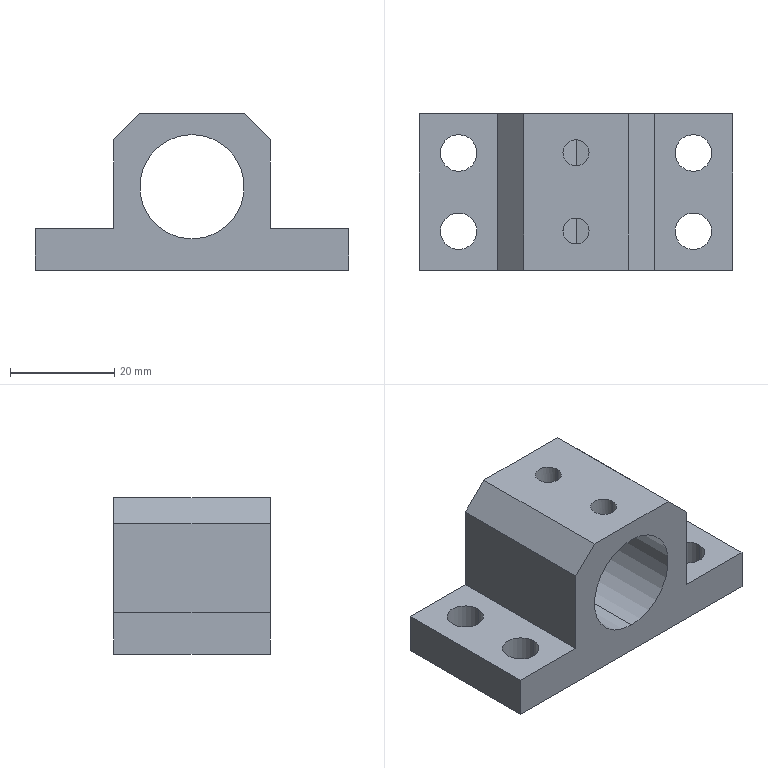Component | SolidWorks | Yk1.5.2AxisSeat-1 | 1 solid | 26 faces | box 60 x 30 x 30 mm | volume 22634 mm3 | cylinder 14 | plane 12 | commonest cylinder face diameters 7 x8 5 x4 20 x2 | material 45
build123d program:
from build123d import *

# Parameters (mm, degrees)
SKETCH1_R                    = 10
BOSS_EXTRUDE1_DEPTH          = 30
F_7_0_7_DIAMETER_HOLE1_D     = 7
F_7_0_7_DIAMETER_HOLE1_DEPTH = 14
F_7_0_7_DIAMETER_HOLE1_TIP   = 2.103
M6_TAPPED_HOLE1_D            = 5
M6_TAPPED_HOLE1_DEPTH        = 8
M6_TAPPED_HOLE1_TIP          = 1.502


with BuildPart() as part:
    # Sketch1 → Boss-Extrude1 (new body)
    with BuildSketch(Plane(origin=(0, 0, 0), x_dir=(1, 0, 0), z_dir=(0, 1, 0))):
        Polygon((-30, 0), (30, 0), (30, -8), (15, -8), (15, -25), (10, -30), (-10, -30), (-15, -25), (-15, -8), (-30, -8), align=None)
        with Locations(Location((0, -16, 0), (0, 0, 270))):
            Circle(SKETCH1_R, mode=Mode.SUBTRACT)
    extrude(amount=BOSS_EXTRUDE1_DEPTH)

    # 7.0 _7_ Diameter Hole1
    with Locations(Plane.XY.offset(8)):
        with Locations((-22.5, 22.5), (-22.5, 7.5), (22.5, 7.5), (22.5, 22.5)):
            Hole(F_7_0_7_DIAMETER_HOLE1_D / 2, depth=F_7_0_7_DIAMETER_HOLE1_DEPTH)
            with Locations((0, 0, -(F_7_0_7_DIAMETER_HOLE1_DEPTH + F_7_0_7_DIAMETER_HOLE1_TIP / 2))):  # 118° drill point
                Cone(0, F_7_0_7_DIAMETER_HOLE1_D / 2, F_7_0_7_DIAMETER_HOLE1_TIP, mode=Mode.SUBTRACT)

    # M6 Tapped Hole1
    with Locations(Plane.XY.offset(30)):
        with Locations((0, 22.5), (0, 7.5)):
            Hole(M6_TAPPED_HOLE1_D / 2, depth=M6_TAPPED_HOLE1_DEPTH)
            with Locations((0, 0, -(M6_TAPPED_HOLE1_DEPTH + M6_TAPPED_HOLE1_TIP / 2))):  # 118° drill point
                Cone(0, M6_TAPPED_HOLE1_D / 2, M6_TAPPED_HOLE1_TIP, mode=Mode.SUBTRACT)


solid = part.part

# Placed as in the assembly
solid = solid.moved(Location((-40.006, 0, 10), (0, 0, 0)))
STEP:
#1=CARTESIAN_POINT('',(-1.575,0.3937,1.417));
#2=VERTEX_POINT('',#1);
#3=CARTESIAN_POINT('',(-1.477,0.2953,1.405));
#4=VERTEX_POINT('',#3);
#5=CARTESIAN_POINT('',(-1.575,0.3937,1.417));
#6=CARTESIAN_POINT('',(-1.569,0.3937,1.417));
#7=CARTESIAN_POINT('',(-1.562,0.3931,1.417));
#8=CARTESIAN_POINT('',(-1.549,0.3905,1.417));
#9=CARTESIAN_POINT('',(-1.543,0.3887,1.416));
#10=CARTESIAN_POINT('',(-1.525,0.3812,1.414));
#11=CARTESIAN_POINT('',(-1.515,0.374,1.413));
#12=CARTESIAN_POINT('',(-1.501,0.3603,1.41));
#13=CARTESIAN_POINT('',(-1.497,0.3553,1.409));
#14=CARTESIAN_POINT('',(-1.49,0.3447,1.408));
#15=CARTESIAN_POINT('',(-1.487,0.3389,1.407));
#16=CARTESIAN_POINT('',(-1.482,0.3271,1.406));
#17=CARTESIAN_POINT('',(-1.48,0.3209,1.406));
#18=CARTESIAN_POINT('',(-1.477,0.3082,1.405));
#19=CARTESIAN_POINT('',(-1.477,0.3017,1.405));
#20=CARTESIAN_POINT('',(-1.477,0.2953,1.405));
#21=B_SPLINE_CURVE_WITH_KNOTS('',3,(#5,#6,#7,#8,#9,#10,#11,#12,#13,#14,#15,#16,#17,#18,#19,#20),.UNSPECIFIED.,.F.,.F.,(4,2,2,2,2,2,2,4),(0.003925,0.004415,0.004905,0.005886,0.006376,0.006867,0.007357,0.007847),.UNSPECIFIED.);
#22=EDGE_CURVE('',#2,#4,#21,.T.);
#23=ORIENTED_EDGE('',*,*,#22,.T.);
#24=CARTESIAN_POINT('',(-1.477,0.2953,1.575));
#25=VERTEX_POINT('',#24);
#26=CARTESIAN_POINT('',(-1.477,0.2953,1.575));
#27=DIRECTION('',(0.,0.,1.));
#28=VECTOR('',#27,39.37);
#29=LINE('',#26,#28);
#30=EDGE_CURVE('',#4,#25,#29,.T.);
#31=ORIENTED_EDGE('',*,*,#30,.T.);
#32=CARTESIAN_POINT('',(-1.673,0.2953,1.575));
#33=VERTEX_POINT('',#32);
#34=CARTESIAN_POINT('',(-1.575,0.2953,1.575));
#35=DIRECTION('',(0.,0.,1.));
#36=DIRECTION('',(-1.,0.,0.));
#37=AXIS2_PLACEMENT_3D('',#34,#35,#36);
#38=CIRCLE('',#37,0.09843);
#39=EDGE_CURVE('',#25,#33,#38,.T.);
#40=ORIENTED_EDGE('',*,*,#39,.T.);
#41=CARTESIAN_POINT('',(-1.673,0.2953,1.405));
#42=VERTEX_POINT('',#41);
#43=CARTESIAN_POINT('',(-1.673,0.2953,1.575));
#44=DIRECTION('',(0.,0.,1.));
#45=VECTOR('',#44,39.37);
#46=LINE('',#43,#45);
#47=EDGE_CURVE('',#42,#33,#46,.T.);
#48=ORIENTED_EDGE('',*,*,#47,.F.);
#49=CARTESIAN_POINT('',(-1.673,0.2953,1.405));
#50=CARTESIAN_POINT('',(-1.673,0.3018,1.405));
#51=CARTESIAN_POINT('',(-1.673,0.3082,1.405));
#52=CARTESIAN_POINT('',(-1.67,0.3208,1.406));
#53=CARTESIAN_POINT('',(-1.668,0.3271,1.406));
#54=CARTESIAN_POINT('',(-1.663,0.339,1.407));
#55=CARTESIAN_POINT('',(-1.66,0.3447,1.408));
#56=CARTESIAN_POINT('',(-1.653,0.3553,1.409));
#57=CARTESIAN_POINT('',(-1.649,0.3604,1.41));
#58=CARTESIAN_POINT('',(-1.636,0.3739,1.413));
#59=CARTESIAN_POINT('',(-1.625,0.3813,1.414));
#60=CARTESIAN_POINT('',(-1.607,0.3886,1.416));
#61=CARTESIAN_POINT('',(-1.601,0.3905,1.417));
#62=CARTESIAN_POINT('',(-1.588,0.3931,1.417));
#63=CARTESIAN_POINT('',(-1.582,0.3937,1.417));
#64=CARTESIAN_POINT('',(-1.575,0.3937,1.417));
#65=B_SPLINE_CURVE_WITH_KNOTS('',3,(#49,#50,#51,#52,#53,#54,#55,#56,#57,#58,#59,#60,#61,#62,#63,#64),.UNSPECIFIED.,.F.,.F.,(4,2,2,2,2,2,2,4),(0.,0.0004906,0.0009812,0.001472,0.001962,0.002944,0.003434,0.003925),.UNSPECIFIED.);
#66=EDGE_CURVE('',#42,#2,#65,.T.);
#67=ORIENTED_EDGE('',*,*,#66,.T.);
#68=EDGE_LOOP('',(#23,#31,#40,#48,#67));
#69=FACE_OUTER_BOUND('',#68,.T.);
#70=CARTESIAN_POINT('',(-1.575,0.2953,1.575));
#71=DIRECTION('',(0.,0.,1.));
#72=DIRECTION('',(-1.,0.,0.));
#73=AXIS2_PLACEMENT_3D('',#70,#71,#72);
#74=CYLINDRICAL_SURFACE('',#73,0.09843);
#75=ADVANCED_FACE('',(#69),#74,.F.);
#76=CARTESIAN_POINT('',(-1.575,0.9843,1.417));
#77=VERTEX_POINT('',#76);
#78=CARTESIAN_POINT('',(-1.477,0.8858,1.405));
#79=VERTEX_POINT('',#78);
#80=CARTESIAN_POINT('',(-1.575,0.9843,1.417));
#81=CARTESIAN_POINT('',(-1.569,0.9843,1.417));
#82=CARTESIAN_POINT('',(-1.562,0.9836,1.417));
#83=CARTESIAN_POINT('',(-1.549,0.9811,1.417));
#84=CARTESIAN_POINT('',(-1.543,0.9792,1.416));
#85=CARTESIAN_POINT('',(-1.525,0.9718,1.414));
#86=CARTESIAN_POINT('',(-1.515,0.9645,1.413));
#87=CARTESIAN_POINT('',(-1.501,0.9508,1.41));
#88=CARTESIAN_POINT('',(-1.497,0.9459,1.409));
#89=CARTESIAN_POINT('',(-1.49,0.9352,1.408));
#90=CARTESIAN_POINT('',(-1.487,0.9295,1.407));
#91=CARTESIAN_POINT('',(-1.482,0.9176,1.406));
#92=CARTESIAN_POINT('',(-1.48,0.9115,1.406));
#93=CARTESIAN_POINT('',(-1.477,0.8988,1.405));
#94=CARTESIAN_POINT('',(-1.477,0.8923,1.405));
#95=CARTESIAN_POINT('',(-1.477,0.8858,1.405));
#96=B_SPLINE_CURVE_WITH_KNOTS('',3,(#80,#81,#82,#83,#84,#85,#86,#87,#88,#89,#90,#91,#92,#93,#94,#95),.UNSPECIFIED.,.F.,.F.,(4,2,2,2,2,2,2,4),(0.003925,0.004415,0.004905,0.005886,0.006376,0.006867,0.007357,0.007847),.UNSPECIFIED.);
#97=EDGE_CURVE('',#77,#79,#96,.T.);
#98=ORIENTED_EDGE('',*,*,#97,.T.);
#99=CARTESIAN_POINT('',(-1.477,0.8858,1.575));
#100=VERTEX_POINT('',#99);
#101=CARTESIAN_POINT('',(-1.477,0.8858,1.575));
#102=DIRECTION('',(0.,0.,1.));
#103=VECTOR('',#102,39.37);
#104=LINE('',#101,#103);
#105=EDGE_CURVE('',#79,#100,#104,.T.);
#106=ORIENTED_EDGE('',*,*,#105,.T.);
#107=CARTESIAN_POINT('',(-1.673,0.8858,1.575));
#108=VERTEX_POINT('',#107);
#109=CARTESIAN_POINT('',(-1.575,0.8858,1.575));
#110=DIRECTION('',(0.,0.,1.));
#111=DIRECTION('',(-1.,0.,0.));
#112=AXIS2_PLACEMENT_3D('',#109,#110,#111);
#113=CIRCLE('',#112,0.09843);
#114=EDGE_CURVE('',#100,#108,#113,.T.);
#115=ORIENTED_EDGE('',*,*,#114,.T.);
#116=CARTESIAN_POINT('',(-1.673,0.8858,1.405));
#117=VERTEX_POINT('',#116);
#118=CARTESIAN_POINT('',(-1.673,0.8858,1.575));
#119=DIRECTION('',(0.,0.,1.));
#120=VECTOR('',#119,39.37);
#121=LINE('',#118,#120);
#122=EDGE_CURVE('',#117,#108,#121,.T.);
#123=ORIENTED_EDGE('',*,*,#122,.F.);
#124=CARTESIAN_POINT('',(-1.673,0.8858,1.405));
#125=CARTESIAN_POINT('',(-1.673,0.8924,1.405));
#126=CARTESIAN_POINT('',(-1.673,0.8988,1.405));
#127=CARTESIAN_POINT('',(-1.67,0.9114,1.406));
#128=CARTESIAN_POINT('',(-1.668,0.9177,1.406));
#129=CARTESIAN_POINT('',(-1.663,0.9296,1.407));
#130=CARTESIAN_POINT('',(-1.66,0.9352,1.408));
#131=CARTESIAN_POINT('',(-1.653,0.9459,1.409));
#132=CARTESIAN_POINT('',(-1.649,0.9509,1.41));
#133=CARTESIAN_POINT('',(-1.636,0.9645,1.413));
#134=CARTESIAN_POINT('',(-1.625,0.9718,1.414));
#135=CARTESIAN_POINT('',(-1.607,0.9792,1.416));
#136=CARTESIAN_POINT('',(-1.601,0.9811,1.417));
#137=CARTESIAN_POINT('',(-1.588,0.9836,1.417));
#138=CARTESIAN_POINT('',(-1.582,0.9843,1.417));
#139=CARTESIAN_POINT('',(-1.575,0.9843,1.417));
#140=B_SPLINE_CURVE_WITH_KNOTS('',3,(#124,#125,#126,#127,#128,#129,#130,#131,#132,#133,#134,#135,#136,#137,#138,#139),.UNSPECIFIED.,.F.,.F.,(4,2,2,2,2,2,2,4),(0.,0.0004906,0.0009812,0.001472,0.001962,0.002944,0.003434,0.003925),.UNSPECIFIED.);
#141=EDGE_CURVE('',#117,#77,#140,.T.);
#142=ORIENTED_EDGE('',*,*,#141,.T.);
#143=EDGE_LOOP('',(#98,#106,#115,#123,#142));
#144=FACE_OUTER_BOUND('',#143,.T.);
#145=CARTESIAN_POINT('',(-1.575,0.8858,1.575));
#146=DIRECTION('',(0.,0.,1.));
#147=DIRECTION('',(-1.,0.,0.));
#148=AXIS2_PLACEMENT_3D('',#145,#146,#147);
#149=CYLINDRICAL_SURFACE('',#148,0.09843);
#150=ADVANCED_FACE('',(#144),#149,.F.);
#151=CARTESIAN_POINT('',(-0.5514,0.2953,0.3937));
#152=VERTEX_POINT('',#151);
#153=CARTESIAN_POINT('',(-0.827,0.2953,0.3937));
#154=VERTEX_POINT('',#153);
#155=CARTESIAN_POINT('',(-0.6892,0.2953,0.3937));
#156=DIRECTION('',(-0.,0.,1.));
#157=DIRECTION('',(-1.,0.,0.));
#158=AXIS2_PLACEMENT_3D('',#155,#156,#157);
#159=CIRCLE('',#158,0.1378);
#160=EDGE_CURVE('',#152,#154,#159,.T.);
#161=ORIENTED_EDGE('',*,*,#160,.F.);
#162=CARTESIAN_POINT('',(-0.5514,0.2953,0.7087));
#163=VERTEX_POINT('',#162);
#164=CARTESIAN_POINT('',(-0.5514,0.2953,0.7087));
#165=DIRECTION('',(0.,0.,1.));
#166=VECTOR('',#165,39.37);
#167=LINE('',#164,#166);
#168=EDGE_CURVE('',#152,#163,#167,.T.);
#169=ORIENTED_EDGE('',*,*,#168,.T.);
#170=CARTESIAN_POINT('',(-0.827,0.2953,0.7087));
#171=VERTEX_POINT('',#170);
#172=CARTESIAN_POINT('',(-0.6892,0.2953,0.7087));
#173=DIRECTION('',(0.,0.,1.));
#174=DIRECTION('',(-1.,0.,0.));
#175=AXIS2_PLACEMENT_3D('',#172,#173,#174);
#176=CIRCLE('',#175,0.1378);
#177=EDGE_CURVE('',#163,#171,#176,.T.);
#178=ORIENTED_EDGE('',*,*,#177,.T.);
#179=CARTESIAN_POINT('',(-0.827,0.2953,0.7087));
#180=DIRECTION('',(0.,0.,1.));
#181=VECTOR('',#180,39.37);
#182=LINE('',#179,#181);
#183=EDGE_CURVE('',#154,#171,#182,.T.);
#184=ORIENTED_EDGE('',*,*,#183,.F.);
#185=EDGE_LOOP('',(#161,#169,#178,#184));
#186=FACE_OUTER_BOUND('',#185,.T.);
#187=CARTESIAN_POINT('',(-0.6892,0.2953,0.7087));
#188=DIRECTION('',(0.,0.,1.));
#189=DIRECTION('',(-1.,0.,0.));
#190=AXIS2_PLACEMENT_3D('',#187,#188,#189);
#191=CYLINDRICAL_SURFACE('',#190,0.1378);
#192=ADVANCED_FACE('',(#186),#191,.F.);
#193=CARTESIAN_POINT('',(-0.5514,0.8858,0.3937));
#194=VERTEX_POINT('',#193);
#195=CARTESIAN_POINT('',(-0.827,0.8858,0.3937));
#196=VERTEX_POINT('',#195);
#197=CARTESIAN_POINT('',(-0.6892,0.8858,0.3937));
#198=DIRECTION('',(-0.,0.,1.));
#199=DIRECTION('',(-1.,0.,0.));
#200=AXIS2_PLACEMENT_3D('',#197,#198,#199);
#201=CIRCLE('',#200,0.1378);
#202=EDGE_CURVE('',#194,#196,#201,.T.);
#203=ORIENTED_EDGE('',*,*,#202,.F.);
#204=CARTESIAN_POINT('',(-0.5514,0.8858,0.7087));
#205=VERTEX_POINT('',#204);
#206=CARTESIAN_POINT('',(-0.5514,0.8858,0.7087));
#207=DIRECTION('',(0.,0.,1.));
#208=VECTOR('',#207,39.37);
#209=LINE('',#206,#208);
#210=EDGE_CURVE('',#194,#205,#209,.T.);
#211=ORIENTED_EDGE('',*,*,#210,.T.);
#212=CARTESIAN_POINT('',(-0.827,0.8858,0.7087));
#213=VERTEX_POINT('',#212);
#214=CARTESIAN_POINT('',(-0.6892,0.8858,0.7087));
#215=DIRECTION('',(0.,0.,1.));
#216=DIRECTION('',(-1.,0.,0.));
#217=AXIS2_PLACEMENT_3D('',#214,#215,#216);
#218=CIRCLE('',#217,0.1378);
#219=EDGE_CURVE('',#205,#213,#218,.T.);
#220=ORIENTED_EDGE('',*,*,#219,.T.);
#221=CARTESIAN_POINT('',(-0.827,0.8858,0.7087));
#222=DIRECTION('',(0.,0.,1.));
#223=VECTOR('',#222,39.37);
#224=LINE('',#221,#223);
#225=EDGE_CURVE('',#196,#213,#224,.T.);
#226=ORIENTED_EDGE('',*,*,#225,.F.);
#227=EDGE_LOOP('',(#203,#211,#220,#226));
#228=FACE_OUTER_BOUND('',#227,.T.);
#229=CARTESIAN_POINT('',(-0.6892,0.8858,0.7087));
#230=DIRECTION('',(0.,0.,1.));
#231=DIRECTION('',(-1.,0.,0.));
#232=AXIS2_PLACEMENT_3D('',#229,#230,#231);
#233=CYLINDRICAL_SURFACE('',#232,0.1378);
#234=ADVANCED_FACE('',(#228),#233,.F.);
#235=CARTESIAN_POINT('',(-2.323,0.8858,0.3937));
#236=VERTEX_POINT('',#235);
#237=CARTESIAN_POINT('',(-2.599,0.8858,0.3937));
#238=VERTEX_POINT('',#237);
#239=CARTESIAN_POINT('',(-2.461,0.8858,0.3937));
#240=DIRECTION('',(-0.,0.,1.));
#241=DIRECTION('',(-1.,0.,0.));
#242=AXIS2_PLACEMENT_3D('',#239,#240,#241);
#243=CIRCLE('',#242,0.1378);
#244=EDGE_CURVE('',#236,#238,#243,.T.);
#245=ORIENTED_EDGE('',*,*,#244,.F.);
#246=CARTESIAN_POINT('',(-2.323,0.8858,0.7087));
#247=VERTEX_POINT('',#246);
#248=CARTESIAN_POINT('',(-2.323,0.8858,0.7087));
#249=DIRECTION('',(0.,0.,1.));
#250=VECTOR('',#249,39.37);
#251=LINE('',#248,#250);
#252=EDGE_CURVE('',#236,#247,#251,.T.);
#253=ORIENTED_EDGE('',*,*,#252,.T.);
#254=CARTESIAN_POINT('',(-2.599,0.8858,0.7087));
#255=VERTEX_POINT('',#254);
#256=CARTESIAN_POINT('',(-2.461,0.8858,0.7087));
#257=DIRECTION('',(0.,0.,1.));
#258=DIRECTION('',(-1.,0.,0.));
#259=AXIS2_PLACEMENT_3D('',#256,#257,#258);
#260=CIRCLE('',#259,0.1378);
#261=EDGE_CURVE('',#247,#255,#260,.T.);
#262=ORIENTED_EDGE('',*,*,#261,.T.);
#263=CARTESIAN_POINT('',(-2.599,0.8858,0.7087));
#264=DIRECTION('',(0.,0.,1.));
#265=VECTOR('',#264,39.37);
#266=LINE('',#263,#265);
#267=EDGE_CURVE('',#238,#255,#266,.T.);
#268=ORIENTED_EDGE('',*,*,#267,.F.);
#269=EDGE_LOOP('',(#245,#253,#262,#268));
#270=FACE_OUTER_BOUND('',#269,.T.);
#271=CARTESIAN_POINT('',(-2.461,0.8858,0.7087));
#272=DIRECTION('',(0.,0.,1.));
#273=DIRECTION('',(-1.,0.,0.));
#274=AXIS2_PLACEMENT_3D('',#271,#272,#273);
#275=CYLINDRICAL_SURFACE('',#274,0.1378);
#276=ADVANCED_FACE('',(#270),#275,.F.);
#277=CARTESIAN_POINT('',(-2.323,0.2953,0.3937));
#278=VERTEX_POINT('',#277);
#279=CARTESIAN_POINT('',(-2.599,0.2953,0.3937));
#280=VERTEX_POINT('',#279);
#281=CARTESIAN_POINT('',(-2.461,0.2953,0.3937));
#282=DIRECTION('',(-0.,0.,1.));
#283=DIRECTION('',(-1.,0.,0.));
#284=AXIS2_PLACEMENT_3D('',#281,#282,#283);
#285=CIRCLE('',#284,0.1378);
#286=EDGE_CURVE('',#278,#280,#285,.T.);
#287=ORIENTED_EDGE('',*,*,#286,.F.);
#288=CARTESIAN_POINT('',(-2.323,0.2953,0.7087));
#289=VERTEX_POINT('',#288);
#290=CARTESIAN_POINT('',(-2.323,0.2953,0.7087));
#291=DIRECTION('',(0.,0.,1.));
#292=VECTOR('',#291,39.37);
#293=LINE('',#290,#292);
#294=EDGE_CURVE('',#278,#289,#293,.T.);
#295=ORIENTED_EDGE('',*,*,#294,.T.);
#296=CARTESIAN_POINT('',(-2.599,0.2953,0.7087));
#297=VERTEX_POINT('',#296);
#298=CARTESIAN_POINT('',(-2.461,0.2953,0.7087));
#299=DIRECTION('',(0.,0.,1.));
#300=DIRECTION('',(-1.,0.,0.));
#301=AXIS2_PLACEMENT_3D('',#298,#299,#300);
#302=CIRCLE('',#301,0.1378);
#303=EDGE_CURVE('',#289,#297,#302,.T.);
#304=ORIENTED_EDGE('',*,*,#303,.T.);
#305=CARTESIAN_POINT('',(-2.599,0.2953,0.7087));
#306=DIRECTION('',(0.,0.,1.));
#307=VECTOR('',#306,39.37);
#308=LINE('',#305,#307);
#309=EDGE_CURVE('',#280,#297,#308,.T.);
#310=ORIENTED_EDGE('',*,*,#309,.F.);
#311=EDGE_LOOP('',(#287,#295,#304,#310));
#312=FACE_OUTER_BOUND('',#311,.T.);
#313=CARTESIAN_POINT('',(-2.461,0.2953,0.7087));
#314=DIRECTION('',(0.,0.,1.));
#315=DIRECTION('',(-1.,0.,0.));
#316=AXIS2_PLACEMENT_3D('',#313,#314,#315);
#317=CYLINDRICAL_SURFACE('',#316,0.1378);
#318=ADVANCED_FACE('',(#312),#317,.F.);
#319=CARTESIAN_POINT('',(-1.575,-0.,0.6299));
#320=VERTEX_POINT('',#319);
#321=CARTESIAN_POINT('',(-1.575,-0.,1.417));
#322=VERTEX_POINT('',#321);
#323=CARTESIAN_POINT('',(-1.575,-0.,1.024));
#324=DIRECTION('',(0.,-1.,-0.));
#325=DIRECTION('',(0.,0.,1.));
#326=AXIS2_PLACEMENT_3D('',#323,#324,#325);
#327=CIRCLE('',#326,0.3937);
#328=EDGE_CURVE('',#320,#322,#327,.T.);
#329=ORIENTED_EDGE('',*,*,#328,.T.);
#330=CARTESIAN_POINT('',(-1.575,0.1969,1.417));
#331=VERTEX_POINT('',#330);
#332=CARTESIAN_POINT('',(-1.575,-0.,1.417));
#333=DIRECTION('',(-0.,1.,0.));
#334=VECTOR('',#333,39.37);
#335=LINE('',#332,#334);
#336=EDGE_CURVE('',#322,#331,#335,.T.);
#337=ORIENTED_EDGE('',*,*,#336,.T.);
#338=CARTESIAN_POINT('',(-1.477,0.2953,1.405));
#339=CARTESIAN_POINT('',(-1.477,0.2824,1.405));
#340=CARTESIAN_POINT('',(-1.479,0.2694,1.406));
#341=CARTESIAN_POINT('',(-1.487,0.2516,1.407));
#342=CARTESIAN_POINT('',(-1.49,0.2459,1.408));
#343=CARTESIAN_POINT('',(-1.497,0.2352,1.409));
#344=CARTESIAN_POINT('',(-1.501,0.2302,1.41));
#345=CARTESIAN_POINT('',(-1.51,0.2212,1.412));
#346=CARTESIAN_POINT('',(-1.515,0.217,1.413));
#347=CARTESIAN_POINT('',(-1.526,0.2099,1.414));
#348=CARTESIAN_POINT('',(-1.531,0.2069,1.415));
#349=CARTESIAN_POINT('',(-1.543,0.2019,1.416));
#350=CARTESIAN_POINT('',(-1.549,0.2,1.417));
#351=CARTESIAN_POINT('',(-1.562,0.1975,1.417));
#352=CARTESIAN_POINT('',(-1.569,0.1969,1.417));
#353=CARTESIAN_POINT('',(-1.575,0.1969,1.417));
#354=B_SPLINE_CURVE_WITH_KNOTS('',3,(#338,#339,#340,#341,#342,#343,#344,#345,#346,#347,#348,#349,#350,#351,#352,#353),.UNSPECIFIED.,.F.,.F.,(4,2,2,2,2,2,2,4),(0.007847,0.008828,0.009319,0.009809,0.0103,0.01079,0.01128,0.01177),.UNSPECIFIED.);
#355=EDGE_CURVE('',#4,#331,#354,.T.);
#356=ORIENTED_EDGE('',*,*,#355,.F.);
#357=ORIENTED_EDGE('',*,*,#22,.F.);
#358=CARTESIAN_POINT('',(-1.575,0.7874,1.417));
#359=VERTEX_POINT('',#358);
#360=CARTESIAN_POINT('',(-1.575,-0.,1.417));
#361=DIRECTION('',(-0.,1.,0.));
#362=VECTOR('',#361,39.37);
#363=LINE('',#360,#362);
#364=EDGE_CURVE('',#2,#359,#363,.T.);
#365=ORIENTED_EDGE('',*,*,#364,.T.);
#366=CARTESIAN_POINT('',(-1.477,0.8858,1.405));
#367=CARTESIAN_POINT('',(-1.477,0.873,1.405));
#368=CARTESIAN_POINT('',(-1.479,0.8599,1.406));
#369=CARTESIAN_POINT('',(-1.487,0.8422,1.407));
#370=CARTESIAN_POINT('',(-1.49,0.8364,1.408));
#371=CARTESIAN_POINT('',(-1.497,0.8257,1.409));
#372=CARTESIAN_POINT('',(-1.501,0.8208,1.41));
#373=CARTESIAN_POINT('',(-1.51,0.8117,1.412));
#374=CARTESIAN_POINT('',(-1.515,0.8076,1.413));
#375=CARTESIAN_POINT('',(-1.526,0.8005,1.414));
#376=CARTESIAN_POINT('',(-1.531,0.7974,1.415));
#377=CARTESIAN_POINT('',(-1.543,0.7925,1.416));
#378=CARTESIAN_POINT('',(-1.549,0.7906,1.417));
#379=CARTESIAN_POINT('',(-1.562,0.7881,1.417));
#380=CARTESIAN_POINT('',(-1.569,0.7874,1.417));
#381=CARTESIAN_POINT('',(-1.575,0.7874,1.417));
#382=B_SPLINE_CURVE_WITH_KNOTS('',3,(#366,#367,#368,#369,#370,#371,#372,#373,#374,#375,#376,#377,#378,#379,#380,#381),.UNSPECIFIED.,.F.,.F.,(4,2,2,2,2,2,2,4),(0.007847,0.008828,0.009319,0.009809,0.0103,0.01079,0.01128,0.01177),.UNSPECIFIED.);
#383=EDGE_CURVE('',#79,#359,#382,.T.);
#384=ORIENTED_EDGE('',*,*,#383,.F.);
#385=ORIENTED_EDGE('',*,*,#97,.F.);
#386=CARTESIAN_POINT('',(-1.575,1.181,1.417));
#387=VERTEX_POINT('',#386);
#388=CARTESIAN_POINT('',(-1.575,-0.,1.417));
#389=DIRECTION('',(-0.,1.,0.));
#390=VECTOR('',#389,39.37);
#391=LINE('',#388,#390);
#392=EDGE_CURVE('',#77,#387,#391,.T.);
#393=ORIENTED_EDGE('',*,*,#392,.T.);
#394=CARTESIAN_POINT('',(-1.575,1.181,0.6299));
#395=VERTEX_POINT('',#394);
#396=CARTESIAN_POINT('',(-1.575,1.181,1.024));
#397=DIRECTION('',(0.,-1.,-0.));
#398=DIRECTION('',(0.,0.,1.));
#399=AXIS2_PLACEMENT_3D('',#396,#397,#398);
#400=CIRCLE('',#399,0.3937);
#401=EDGE_CURVE('',#395,#387,#400,.T.);
#402=ORIENTED_EDGE('',*,*,#401,.F.);
#403=CARTESIAN_POINT('',(-1.575,-0.,0.6299));
#404=DIRECTION('',(-0.,1.,0.));
#405=VECTOR('',#404,39.37);
#406=LINE('',#403,#405);
#407=EDGE_CURVE('',#320,#395,#406,.T.);
#408=ORIENTED_EDGE('',*,*,#407,.F.);
#409=EDGE_LOOP('',(#329,#337,#356,#357,#365,#384,#385,#393,#402,#408));
#410=FACE_OUTER_BOUND('',#409,.T.);
#411=CARTESIAN_POINT('',(-1.575,-0.,1.024));
#412=DIRECTION('',(-0.,1.,0.));
#413=DIRECTION('',(0.,0.,-1.));
#414=AXIS2_PLACEMENT_3D('',#411,#412,#413);
#415=CYLINDRICAL_SURFACE('',#414,0.3937);
#416=ADVANCED_FACE('',(#410),#415,.F.);
#417=CARTESIAN_POINT('',(-0.394,-0.,0.3937));
#418=VERTEX_POINT('',#417);
#419=CARTESIAN_POINT('',(-0.394,-0.,0.7087));
#420=VERTEX_POINT('',#419);
#421=CARTESIAN_POINT('',(-0.394,-0.,0.3937));
#422=DIRECTION('',(0.,0.,1.));
#423=VECTOR('',#422,39.37);
#424=LINE('',#421,#423);
#425=EDGE_CURVE('',#418,#420,#424,.T.);
#426=ORIENTED_EDGE('',*,*,#425,.T.);
#427=CARTESIAN_POINT('',(-0.9845,-0.,0.7087));
#428=VERTEX_POINT('',#427);
#429=CARTESIAN_POINT('',(-0.394,-0.,0.7087));
#430=DIRECTION('',(-1.,0.,-0.));
#431=VECTOR('',#430,39.37);
#432=LINE('',#429,#431);
#433=EDGE_CURVE('',#420,#428,#432,.T.);
#434=ORIENTED_EDGE('',*,*,#433,.T.);
#435=CARTESIAN_POINT('',(-0.9845,-0.,1.378));
#436=VERTEX_POINT('',#435);
#437=CARTESIAN_POINT('',(-0.9845,-0.,0.7087));
#438=DIRECTION('',(0.,0.,1.));
#439=VECTOR('',#438,39.37);
#440=LINE('',#437,#439);
#441=EDGE_CURVE('',#428,#436,#440,.T.);
#442=ORIENTED_EDGE('',*,*,#441,.T.);
#443=CARTESIAN_POINT('',(-1.181,-0.,1.575));
#444=VERTEX_POINT('',#443);
#445=CARTESIAN_POINT('',(-0.9845,-0.,1.378));
#446=DIRECTION('',(-0.7071,0.,0.7071));
#447=VECTOR('',#446,39.37);
#448=LINE('',#445,#447);
#449=EDGE_CURVE('',#436,#444,#448,.T.);
#450=ORIENTED_EDGE('',*,*,#449,.T.);
#451=CARTESIAN_POINT('',(-1.969,-0.,1.575));
#452=VERTEX_POINT('',#451);
#453=CARTESIAN_POINT('',(-1.969,-0.,1.575));
#454=DIRECTION('',(-1.,0.,-0.));
#455=VECTOR('',#454,39.37);
#456=LINE('',#453,#455);
#457=EDGE_CURVE('',#444,#452,#456,.T.);
#458=ORIENTED_EDGE('',*,*,#457,.T.);
#459=CARTESIAN_POINT('',(-2.166,-0.,1.378));
#460=VERTEX_POINT('',#459);
#461=CARTESIAN_POINT('',(-2.166,-0.,1.378));
#462=DIRECTION('',(-0.7071,0.,-0.7071));
#463=VECTOR('',#462,39.37);
#464=LINE('',#461,#463);
#465=EDGE_CURVE('',#452,#460,#464,.T.);
#466=ORIENTED_EDGE('',*,*,#465,.T.);
#467=CARTESIAN_POINT('',(-2.166,-0.,0.7087));
#468=VERTEX_POINT('',#467);
#469=CARTESIAN_POINT('',(-2.166,-0.,0.7087));
#470=DIRECTION('',(0.,-0.,-1.));
#471=VECTOR('',#470,39.37);
#472=LINE('',#469,#471);
#473=EDGE_CURVE('',#460,#468,#472,.T.);
#474=ORIENTED_EDGE('',*,*,#473,.T.);
#475=CARTESIAN_POINT('',(-2.756,-0.,0.7087));
#476=VERTEX_POINT('',#475);
#477=CARTESIAN_POINT('',(-2.756,-0.,0.7087));
#478=DIRECTION('',(-1.,0.,-0.));
#479=VECTOR('',#478,39.37);
#480=LINE('',#477,#479);
#481=EDGE_CURVE('',#468,#476,#480,.T.);
#482=ORIENTED_EDGE('',*,*,#481,.T.);
#483=CARTESIAN_POINT('',(-2.756,-0.,0.3937));
#484=VERTEX_POINT('',#483);
#485=CARTESIAN_POINT('',(-2.756,-0.,0.3937));
#486=DIRECTION('',(-0.,-0.,-1.));
#487=VECTOR('',#486,39.37);
#488=LINE('',#485,#487);
#489=EDGE_CURVE('',#476,#484,#488,.T.);
#490=ORIENTED_EDGE('',*,*,#489,.T.);
#491=CARTESIAN_POINT('',(-0.394,-0.,0.3937));
#492=DIRECTION('',(1.,-0.,0.));
#493=VECTOR('',#492,39.37);
#494=LINE('',#491,#493);
#495=EDGE_CURVE('',#484,#418,#494,.T.);
#496=ORIENTED_EDGE('',*,*,#495,.T.);
#497=EDGE_LOOP('',(#426,#434,#442,#450,#458,#466,#474,#482,#490,#496));
#498=FACE_OUTER_BOUND('',#497,.T.);
#499=ORIENTED_EDGE('',*,*,#328,.F.);
#500=CARTESIAN_POINT('',(-1.575,-0.,1.024));
#501=DIRECTION('',(0.,-1.,-0.));
#502=DIRECTION('',(0.,0.,1.));
#503=AXIS2_PLACEMENT_3D('',#500,#501,#502);
#504=CIRCLE('',#503,0.3937);
#505=EDGE_CURVE('',#322,#320,#504,.T.);
#506=ORIENTED_EDGE('',*,*,#505,.F.);
#507=EDGE_LOOP('',(#499,#506));
#508=FACE_BOUND('',#507,.T.);
#509=CARTESIAN_POINT('',(-1.575,-0.,0.3937));
#510=DIRECTION('',(0.,-1.,0.));
#511=DIRECTION('',(0.,0.,1.));
#512=AXIS2_PLACEMENT_3D('',#509,#510,#511);
#513=PLANE('',#512);
#514=ADVANCED_FACE('',(#498,#508),#513,.T.);
#515=CARTESIAN_POINT('',(-0.394,1.181,0.3937));
#516=VERTEX_POINT('',#515);
#517=CARTESIAN_POINT('',(-0.394,1.181,0.7087));
#518=VERTEX_POINT('',#517);
#519=CARTESIAN_POINT('',(-0.394,1.181,0.3937));
#520=DIRECTION('',(0.,0.,1.));
#521=VECTOR('',#520,39.37);
#522=LINE('',#519,#521);
#523=EDGE_CURVE('',#516,#518,#522,.T.);
#524=ORIENTED_EDGE('',*,*,#523,.F.);
#525=CARTESIAN_POINT('',(-2.756,1.181,0.3937));
#526=VERTEX_POINT('',#525);
#527=CARTESIAN_POINT('',(-0.394,1.181,0.3937));
#528=DIRECTION('',(1.,-0.,0.));
#529=VECTOR('',#528,39.37);
#530=LINE('',#527,#529);
#531=EDGE_CURVE('',#526,#516,#530,.T.);
#532=ORIENTED_EDGE('',*,*,#531,.F.);
#533=CARTESIAN_POINT('',(-2.756,1.181,0.7087));
#534=VERTEX_POINT('',#533);
#535=CARTESIAN_POINT('',(-2.756,1.181,0.3937));
#536=DIRECTION('',(-0.,-0.,-1.));
#537=VECTOR('',#536,39.37);
#538=LINE('',#535,#537);
#539=EDGE_CURVE('',#534,#526,#538,.T.);
#540=ORIENTED_EDGE('',*,*,#539,.F.);
#541=CARTESIAN_POINT('',(-2.166,1.181,0.7087));
#542=VERTEX_POINT('',#541);
#543=CARTESIAN_POINT('',(-2.756,1.181,0.7087));
#544=DIRECTION('',(-1.,0.,-0.));
#545=VECTOR('',#544,39.37);
#546=LINE('',#543,#545);
#547=EDGE_CURVE('',#542,#534,#546,.T.);
#548=ORIENTED_EDGE('',*,*,#547,.F.);
#549=CARTESIAN_POINT('',(-2.166,1.181,1.378));
#550=VERTEX_POINT('',#549);
#551=CARTESIAN_POINT('',(-2.166,1.181,0.7087));
#552=DIRECTION('',(0.,-0.,-1.));
#553=VECTOR('',#552,39.37);
#554=LINE('',#551,#553);
#555=EDGE_CURVE('',#550,#542,#554,.T.);
#556=ORIENTED_EDGE('',*,*,#555,.F.);
#557=CARTESIAN_POINT('',(-1.969,1.181,1.575));
#558=VERTEX_POINT('',#557);
#559=CARTESIAN_POINT('',(-2.166,1.181,1.378));
#560=DIRECTION('',(-0.7071,0.,-0.7071));
#561=VECTOR('',#560,39.37);
#562=LINE('',#559,#561);
#563=EDGE_CURVE('',#558,#550,#562,.T.);
#564=ORIENTED_EDGE('',*,*,#563,.F.);
#565=CARTESIAN_POINT('',(-1.181,1.181,1.575));
#566=VERTEX_POINT('',#565);
#567=CARTESIAN_POINT('',(-1.969,1.181,1.575));
#568=DIRECTION('',(-1.,0.,-0.));
#569=VECTOR('',#568,39.37);
#570=LINE('',#567,#569);
#571=EDGE_CURVE('',#566,#558,#570,.T.);
#572=ORIENTED_EDGE('',*,*,#571,.F.);
#573=CARTESIAN_POINT('',(-0.9845,1.181,1.378));
#574=VERTEX_POINT('',#573);
#575=CARTESIAN_POINT('',(-0.9845,1.181,1.378));
#576=DIRECTION('',(-0.7071,0.,0.7071));
#577=VECTOR('',#576,39.37);
#578=LINE('',#575,#577);
#579=EDGE_CURVE('',#574,#566,#578,.T.);
#580=ORIENTED_EDGE('',*,*,#579,.F.);
#581=CARTESIAN_POINT('',(-0.9845,1.181,0.7087));
#582=VERTEX_POINT('',#581);
#583=CARTESIAN_POINT('',(-0.9845,1.181,0.7087));
#584=DIRECTION('',(0.,0.,1.));
#585=VECTOR('',#584,39.37);
#586=LINE('',#583,#585);
#587=EDGE_CURVE('',#582,#574,#586,.T.);
#588=ORIENTED_EDGE('',*,*,#587,.F.);
#589=CARTESIAN_POINT('',(-0.394,1.181,0.7087));
#590=DIRECTION('',(-1.,0.,-0.));
#591=VECTOR('',#590,39.37);
#592=LINE('',#589,#591);
#593=EDGE_CURVE('',#518,#582,#592,.T.);
#594=ORIENTED_EDGE('',*,*,#593,.F.);
#595=EDGE_LOOP('',(#524,#532,#540,#548,#556,#564,#572,#580,#588,#594));
#596=FACE_OUTER_BOUND('',#595,.T.);
#597=ORIENTED_EDGE('',*,*,#401,.T.);
#598=CARTESIAN_POINT('',(-1.575,1.181,1.024));
#599=DIRECTION('',(0.,-1.,-0.));
#600=DIRECTION('',(0.,0.,1.));
#601=AXIS2_PLACEMENT_3D('',#598,#599,#600);
#602=CIRCLE('',#601,0.3937);
#603=EDGE_CURVE('',#387,#395,#602,.T.);
#604=ORIENTED_EDGE('',*,*,#603,.T.);
#605=EDGE_LOOP('',(#597,#604));
#606=FACE_BOUND('',#605,.T.);
#607=CARTESIAN_POINT('',(-1.575,1.181,0.3937));
#608=DIRECTION('',(0.,-1.,0.));
#609=DIRECTION('',(0.,0.,1.));
#610=AXIS2_PLACEMENT_3D('',#607,#608,#609);
#611=PLANE('',#610);
#612=ADVANCED_FACE('',(#596,#606),#611,.F.);
#613=ORIENTED_EDGE('',*,*,#523,.T.);
#614=CARTESIAN_POINT('',(-0.394,-0.,0.7087));
#615=DIRECTION('',(-0.,1.,0.));
#616=VECTOR('',#615,39.37);
#617=LINE('',#614,#616);
#618=EDGE_CURVE('',#420,#518,#617,.T.);
#619=ORIENTED_EDGE('',*,*,#618,.F.);
#620=ORIENTED_EDGE('',*,*,#425,.F.);
#621=CARTESIAN_POINT('',(-0.394,-0.,0.3937));
#622=DIRECTION('',(-0.,1.,0.));
#623=VECTOR('',#622,39.37);
#624=LINE('',#621,#623);
#625=EDGE_CURVE('',#418,#516,#624,.T.);
#626=ORIENTED_EDGE('',*,*,#625,.T.);
#627=EDGE_LOOP('',(#613,#619,#620,#626));
#628=FACE_OUTER_BOUND('',#627,.T.);
#629=CARTESIAN_POINT('',(-0.394,-0.,0.3937));
#630=DIRECTION('',(-1.,0.,0.));
#631=DIRECTION('',(-0.,-0.,-1.));
#632=AXIS2_PLACEMENT_3D('',#629,#630,#631);
#633=PLANE('',#632);
#634=ADVANCED_FACE('',(#628),#633,.F.);
#635=CARTESIAN_POINT('',(-0.6892,0.2953,0.7087));
#636=DIRECTION('',(0.,0.,1.));
#637=DIRECTION('',(-1.,0.,0.));
#638=AXIS2_PLACEMENT_3D('',#635,#636,#637);
#639=CIRCLE('',#638,0.1378);
#640=EDGE_CURVE('',#171,#163,#639,.T.);
#641=ORIENTED_EDGE('',*,*,#640,.F.);
#642=ORIENTED_EDGE('',*,*,#177,.F.);
#643=EDGE_LOOP('',(#641,#642));
#644=FACE_BOUND('',#643,.T.);
#645=CARTESIAN_POINT('',(-0.6892,0.8858,0.7087));
#646=DIRECTION('',(0.,0.,1.));
#647=DIRECTION('',(-1.,0.,0.));
#648=AXIS2_PLACEMENT_3D('',#645,#646,#647);
#649=CIRCLE('',#648,0.1378);
#650=EDGE_CURVE('',#213,#205,#649,.T.);
#651=ORIENTED_EDGE('',*,*,#650,.F.);
#652=ORIENTED_EDGE('',*,*,#219,.F.);
#653=EDGE_LOOP('',(#651,#652));
#654=FACE_BOUND('',#653,.T.);
#655=ORIENTED_EDGE('',*,*,#593,.T.);
#656=CARTESIAN_POINT('',(-0.9845,-0.,0.7087));
#657=DIRECTION('',(-0.,1.,0.));
#658=VECTOR('',#657,39.37);
#659=LINE('',#656,#658);
#660=EDGE_CURVE('',#428,#582,#659,.T.);
#661=ORIENTED_EDGE('',*,*,#660,.F.);
#662=ORIENTED_EDGE('',*,*,#433,.F.);
#663=ORIENTED_EDGE('',*,*,#618,.T.);
#664=EDGE_LOOP('',(#655,#661,#662,#663));
#665=FACE_OUTER_BOUND('',#664,.T.);
#666=CARTESIAN_POINT('',(-0.394,-0.,0.7087));
#667=DIRECTION('',(0.,-0.,-1.));
#668=DIRECTION('',(1.,-0.,0.));
#669=AXIS2_PLACEMENT_3D('',#666,#667,#668);
#670=PLANE('',#669);
#671=ADVANCED_FACE('',(#644,#654,#665),#670,.F.);
#672=ORIENTED_EDGE('',*,*,#587,.T.);
#673=CARTESIAN_POINT('',(-0.9845,-0.,1.378));
#674=DIRECTION('',(-0.,1.,0.));
#675=VECTOR('',#674,39.37);
#676=LINE('',#673,#675);
#677=EDGE_CURVE('',#436,#574,#676,.T.);
#678=ORIENTED_EDGE('',*,*,#677,.F.);
#679=ORIENTED_EDGE('',*,*,#441,.F.);
#680=ORIENTED_EDGE('',*,*,#660,.T.);
#681=EDGE_LOOP('',(#672,#678,#679,#680));
#682=FACE_OUTER_BOUND('',#681,.T.);
#683=CARTESIAN_POINT('',(-0.9845,-0.,0.7087));
#684=DIRECTION('',(-1.,0.,0.));
#685=DIRECTION('',(-0.,-0.,-1.));
#686=AXIS2_PLACEMENT_3D('',#683,#684,#685);
#687=PLANE('',#686);
#688=ADVANCED_FACE('',(#682),#687,.F.);
#689=ORIENTED_EDGE('',*,*,#579,.T.);
#690=CARTESIAN_POINT('',(-1.181,-0.,1.575));
#691=DIRECTION('',(-0.,1.,0.));
#692=VECTOR('',#691,39.37);
#693=LINE('',#690,#692);
#694=EDGE_CURVE('',#444,#566,#693,.T.);
#695=ORIENTED_EDGE('',*,*,#694,.F.);
#696=ORIENTED_EDGE('',*,*,#449,.F.);
#697=ORIENTED_EDGE('',*,*,#677,.T.);
#698=EDGE_LOOP('',(#689,#695,#696,#697));
#699=FACE_OUTER_BOUND('',#698,.T.);
#700=CARTESIAN_POINT('',(-0.9845,-0.,1.378));
#701=DIRECTION('',(-0.7071,0.,-0.7071));
#702=DIRECTION('',(0.7071,-0.,-0.7071));
#703=AXIS2_PLACEMENT_3D('',#700,#701,#702);
#704=PLANE('',#703);
#705=ADVANCED_FACE('',(#699),#704,.F.);
#706=CARTESIAN_POINT('',(-1.575,0.2953,1.575));
#707=DIRECTION('',(0.,0.,1.));
#708=DIRECTION('',(-1.,0.,0.));
#709=AXIS2_PLACEMENT_3D('',#706,#707,#708);
#710=CIRCLE('',#709,0.09843);
#711=EDGE_CURVE('',#33,#25,#710,.T.);
#712=ORIENTED_EDGE('',*,*,#711,.F.);
#713=ORIENTED_EDGE('',*,*,#39,.F.);
#714=EDGE_LOOP('',(#712,#713));
#715=FACE_BOUND('',#714,.T.);
#716=CARTESIAN_POINT('',(-1.575,0.8858,1.575));
#717=DIRECTION('',(0.,0.,1.));
#718=DIRECTION('',(-1.,0.,0.));
#719=AXIS2_PLACEMENT_3D('',#716,#717,#718);
#720=CIRCLE('',#719,0.09843);
#721=EDGE_CURVE('',#108,#100,#720,.T.);
#722=ORIENTED_EDGE('',*,*,#721,.F.);
#723=ORIENTED_EDGE('',*,*,#114,.F.);
#724=EDGE_LOOP('',(#722,#723));
#725=FACE_BOUND('',#724,.T.);
#726=ORIENTED_EDGE('',*,*,#571,.T.);
#727=CARTESIAN_POINT('',(-1.969,-0.,1.575));
#728=DIRECTION('',(-0.,1.,0.));
#729=VECTOR('',#728,39.37);
#730=LINE('',#727,#729);
#731=EDGE_CURVE('',#452,#558,#730,.T.);
#732=ORIENTED_EDGE('',*,*,#731,.F.);
#733=ORIENTED_EDGE('',*,*,#457,.F.);
#734=ORIENTED_EDGE('',*,*,#694,.T.);
#735=EDGE_LOOP('',(#726,#732,#733,#734));
#736=FACE_OUTER_BOUND('',#735,.T.);
#737=CARTESIAN_POINT('',(-1.969,-0.,1.575));
#738=DIRECTION('',(0.,-0.,-1.));
#739=DIRECTION('',(1.,-0.,0.));
#740=AXIS2_PLACEMENT_3D('',#737,#738,#739);
#741=PLANE('',#740);
#742=ADVANCED_FACE('',(#715,#725,#736),#741,.F.);
#743=ORIENTED_EDGE('',*,*,#563,.T.);
#744=CARTESIAN_POINT('',(-2.166,-0.,1.378));
#745=DIRECTION('',(-0.,1.,0.));
#746=VECTOR('',#745,39.37);
#747=LINE('',#744,#746);
#748=EDGE_CURVE('',#460,#550,#747,.T.);
#749=ORIENTED_EDGE('',*,*,#748,.F.);
#750=ORIENTED_EDGE('',*,*,#465,.F.);
#751=ORIENTED_EDGE('',*,*,#731,.T.);
#752=EDGE_LOOP('',(#743,#749,#750,#751));
#753=FACE_OUTER_BOUND('',#752,.T.);
#754=CARTESIAN_POINT('',(-2.166,-0.,1.378));
#755=DIRECTION('',(0.7071,-0.,-0.7071));
#756=DIRECTION('',(0.7071,-0.,0.7071));
#757=AXIS2_PLACEMENT_3D('',#754,#755,#756);
#758=PLANE('',#757);
#759=ADVANCED_FACE('',(#753),#758,.F.);
#760=ORIENTED_EDGE('',*,*,#555,.T.);
#761=CARTESIAN_POINT('',(-2.166,-0.,0.7087));
#762=DIRECTION('',(-0.,1.,0.));
#763=VECTOR('',#762,39.37);
#764=LINE('',#761,#763);
#765=EDGE_CURVE('',#468,#542,#764,.T.);
#766=ORIENTED_EDGE('',*,*,#765,.F.);
#767=ORIENTED_EDGE('',*,*,#473,.F.);
#768=ORIENTED_EDGE('',*,*,#748,.T.);
#769=EDGE_LOOP('',(#760,#766,#767,#768));
#770=FACE_OUTER_BOUND('',#769,.T.);
#771=CARTESIAN_POINT('',(-2.166,-0.,0.7087));
#772=DIRECTION('',(1.,-0.,0.));
#773=DIRECTION('',(-0.,0.,1.));
#774=AXIS2_PLACEMENT_3D('',#771,#772,#773);
#775=PLANE('',#774);
#776=ADVANCED_FACE('',(#770),#775,.F.);
#777=CARTESIAN_POINT('',(-2.461,0.8858,0.7087));
#778=DIRECTION('',(0.,0.,1.));
#779=DIRECTION('',(-1.,0.,0.));
#780=AXIS2_PLACEMENT_3D('',#777,#778,#779);
#781=CIRCLE('',#780,0.1378);
#782=EDGE_CURVE('',#255,#247,#781,.T.);
#783=ORIENTED_EDGE('',*,*,#782,.F.);
#784=ORIENTED_EDGE('',*,*,#261,.F.);
#785=EDGE_LOOP('',(#783,#784));
#786=FACE_BOUND('',#785,.T.);
#787=CARTESIAN_POINT('',(-2.461,0.2953,0.7087));
#788=DIRECTION('',(0.,0.,1.));
#789=DIRECTION('',(-1.,0.,0.));
#790=AXIS2_PLACEMENT_3D('',#787,#788,#789);
#791=CIRCLE('',#790,0.1378);
#792=EDGE_CURVE('',#297,#289,#791,.T.);
#793=ORIENTED_EDGE('',*,*,#792,.F.);
#794=ORIENTED_EDGE('',*,*,#303,.F.);
#795=EDGE_LOOP('',(#793,#794));
#796=FACE_BOUND('',#795,.T.);
#797=ORIENTED_EDGE('',*,*,#547,.T.);
#798=CARTESIAN_POINT('',(-2.756,-0.,0.7087));
#799=DIRECTION('',(-0.,1.,0.));
#800=VECTOR('',#799,39.37);
#801=LINE('',#798,#800);
#802=EDGE_CURVE('',#476,#534,#801,.T.);
#803=ORIENTED_EDGE('',*,*,#802,.F.);
#804=ORIENTED_EDGE('',*,*,#481,.F.);
#805=ORIENTED_EDGE('',*,*,#765,.T.);
#806=EDGE_LOOP('',(#797,#803,#804,#805));
#807=FACE_OUTER_BOUND('',#806,.T.);
#808=CARTESIAN_POINT('',(-2.756,-0.,0.7087));
#809=DIRECTION('',(0.,-0.,-1.));
#810=DIRECTION('',(1.,-0.,0.));
#811=AXIS2_PLACEMENT_3D('',#808,#809,#810);
#812=PLANE('',#811);
#813=ADVANCED_FACE('',(#786,#796,#807),#812,.F.);
#814=ORIENTED_EDGE('',*,*,#539,.T.);
#815=CARTESIAN_POINT('',(-2.756,-0.,0.3937));
#816=DIRECTION('',(-0.,1.,0.));
#817=VECTOR('',#816,39.37);
#818=LINE('',#815,#817);
#819=EDGE_CURVE('',#484,#526,#818,.T.);
#820=ORIENTED_EDGE('',*,*,#819,.F.);
#821=ORIENTED_EDGE('',*,*,#489,.F.);
#822=ORIENTED_EDGE('',*,*,#802,.T.);
#823=EDGE_LOOP('',(#814,#820,#821,#822));
#824=FACE_OUTER_BOUND('',#823,.T.);
#825=CARTESIAN_POINT('',(-2.756,-0.,0.3937));
#826=DIRECTION('',(1.,-0.,-0.));
#827=DIRECTION('',(0.,0.,1.));
#828=AXIS2_PLACEMENT_3D('',#825,#826,#827);
#829=PLANE('',#828);
#830=ADVANCED_FACE('',(#824),#829,.F.);
#831=CARTESIAN_POINT('',(-0.6892,0.2953,0.3937));
#832=DIRECTION('',(-0.,0.,1.));
#833=DIRECTION('',(-1.,0.,0.));
#834=AXIS2_PLACEMENT_3D('',#831,#832,#833);
#835=CIRCLE('',#834,0.1378);
#836=EDGE_CURVE('',#154,#152,#835,.T.);
#837=ORIENTED_EDGE('',*,*,#836,.T.);
#838=ORIENTED_EDGE('',*,*,#160,.T.);
#839=EDGE_LOOP('',(#837,#838));
#840=FACE_BOUND('',#839,.T.);
#841=CARTESIAN_POINT('',(-0.6892,0.8858,0.3937));
#842=DIRECTION('',(-0.,0.,1.));
#843=DIRECTION('',(-1.,0.,0.));
#844=AXIS2_PLACEMENT_3D('',#841,#842,#843);
#845=CIRCLE('',#844,0.1378);
#846=EDGE_CURVE('',#196,#194,#845,.T.);
#847=ORIENTED_EDGE('',*,*,#846,.T.);
#848=ORIENTED_EDGE('',*,*,#202,.T.);
#849=EDGE_LOOP('',(#847,#848));
#850=FACE_BOUND('',#849,.T.);
#851=CARTESIAN_POINT('',(-2.461,0.8858,0.3937));
#852=DIRECTION('',(-0.,0.,1.));
#853=DIRECTION('',(-1.,0.,0.));
#854=AXIS2_PLACEMENT_3D('',#851,#852,#853);
#855=CIRCLE('',#854,0.1378);
#856=EDGE_CURVE('',#238,#236,#855,.T.);
#857=ORIENTED_EDGE('',*,*,#856,.T.);
#858=ORIENTED_EDGE('',*,*,#244,.T.);
#859=EDGE_LOOP('',(#857,#858));
#860=FACE_BOUND('',#859,.T.);
#861=CARTESIAN_POINT('',(-2.461,0.2953,0.3937));
#862=DIRECTION('',(-0.,0.,1.));
#863=DIRECTION('',(-1.,0.,0.));
#864=AXIS2_PLACEMENT_3D('',#861,#862,#863);
#865=CIRCLE('',#864,0.1378);
#866=EDGE_CURVE('',#280,#278,#865,.T.);
#867=ORIENTED_EDGE('',*,*,#866,.T.);
#868=ORIENTED_EDGE('',*,*,#286,.T.);
#869=EDGE_LOOP('',(#867,#868));
#870=FACE_BOUND('',#869,.T.);
#871=ORIENTED_EDGE('',*,*,#531,.T.);
#872=ORIENTED_EDGE('',*,*,#625,.F.);
#873=ORIENTED_EDGE('',*,*,#495,.F.);
#874=ORIENTED_EDGE('',*,*,#819,.T.);
#875=EDGE_LOOP('',(#871,#872,#873,#874));
#876=FACE_OUTER_BOUND('',#875,.T.);
#877=CARTESIAN_POINT('',(-0.394,-0.,0.3937));
#878=DIRECTION('',(-0.,0.,1.));
#879=DIRECTION('',(-1.,0.,-0.));
#880=AXIS2_PLACEMENT_3D('',#877,#878,#879);
#881=PLANE('',#880);
#882=ADVANCED_FACE('',(#840,#850,#860,#870,#876),#881,.F.);
#883=ORIENTED_EDGE('',*,*,#336,.F.);
#884=ORIENTED_EDGE('',*,*,#505,.T.);
#885=ORIENTED_EDGE('',*,*,#407,.T.);
#886=ORIENTED_EDGE('',*,*,#603,.F.);
#887=ORIENTED_EDGE('',*,*,#392,.F.);
#888=ORIENTED_EDGE('',*,*,#141,.F.);
#889=CARTESIAN_POINT('',(-1.575,0.7874,1.417));
#890=CARTESIAN_POINT('',(-1.582,0.7874,1.417));
#891=CARTESIAN_POINT('',(-1.588,0.788,1.417));
#892=CARTESIAN_POINT('',(-1.601,0.7906,1.417));
#893=CARTESIAN_POINT('',(-1.607,0.7925,1.416));
#894=CARTESIAN_POINT('',(-1.619,0.7974,1.415));
#895=CARTESIAN_POINT('',(-1.624,0.8004,1.414));
#896=CARTESIAN_POINT('',(-1.635,0.8076,1.413));
#897=CARTESIAN_POINT('',(-1.64,0.8117,1.412));
#898=CARTESIAN_POINT('',(-1.649,0.8207,1.41));
#899=CARTESIAN_POINT('',(-1.653,0.8257,1.409));
#900=CARTESIAN_POINT('',(-1.66,0.8364,1.408));
#901=CARTESIAN_POINT('',(-1.663,0.8421,1.407));
#902=CARTESIAN_POINT('',(-1.668,0.8539,1.406));
#903=CARTESIAN_POINT('',(-1.67,0.8602,1.406));
#904=CARTESIAN_POINT('',(-1.673,0.8729,1.405));
#905=CARTESIAN_POINT('',(-1.673,0.8793,1.405));
#906=CARTESIAN_POINT('',(-1.673,0.8858,1.405));
#907=B_SPLINE_CURVE_WITH_KNOTS('',3,(#889,#890,#891,#892,#893,#894,#895,#896,#897,#898,#899,#900,#901,#902,#903,#904,#905,#906),.UNSPECIFIED.,.F.,.F.,(4,2,2,2,2,2,2,2,4),(0.01177,0.01226,0.01275,0.01324,0.01373,0.01422,0.01471,0.0152,0.01569),.UNSPECIFIED.);
#908=EDGE_CURVE('',#359,#117,#907,.T.);
#909=ORIENTED_EDGE('',*,*,#908,.F.);
#910=ORIENTED_EDGE('',*,*,#364,.F.);
#911=ORIENTED_EDGE('',*,*,#66,.F.);
#912=CARTESIAN_POINT('',(-1.575,0.1969,1.417));
#913=CARTESIAN_POINT('',(-1.582,0.1969,1.417));
#914=CARTESIAN_POINT('',(-1.588,0.1975,1.417));
#915=CARTESIAN_POINT('',(-1.601,0.2,1.417));
#916=CARTESIAN_POINT('',(-1.607,0.2019,1.416));
#917=CARTESIAN_POINT('',(-1.619,0.2068,1.415));
#918=CARTESIAN_POINT('',(-1.624,0.2099,1.414));
#919=CARTESIAN_POINT('',(-1.635,0.217,1.413));
#920=CARTESIAN_POINT('',(-1.64,0.2211,1.412));
#921=CARTESIAN_POINT('',(-1.649,0.2302,1.41));
#922=CARTESIAN_POINT('',(-1.653,0.2352,1.409));
#923=CARTESIAN_POINT('',(-1.66,0.2459,1.408));
#924=CARTESIAN_POINT('',(-1.663,0.2515,1.407));
#925=CARTESIAN_POINT('',(-1.668,0.2634,1.406));
#926=CARTESIAN_POINT('',(-1.67,0.2696,1.406));
#927=CARTESIAN_POINT('',(-1.673,0.2823,1.405));
#928=CARTESIAN_POINT('',(-1.673,0.2887,1.405));
#929=CARTESIAN_POINT('',(-1.673,0.2953,1.405));
#930=B_SPLINE_CURVE_WITH_KNOTS('',3,(#912,#913,#914,#915,#916,#917,#918,#919,#920,#921,#922,#923,#924,#925,#926,#927,#928,#929),.UNSPECIFIED.,.F.,.F.,(4,2,2,2,2,2,2,2,4),(0.01177,0.01226,0.01275,0.01324,0.01373,0.01422,0.01471,0.0152,0.01569),.UNSPECIFIED.);
#931=EDGE_CURVE('',#331,#42,#930,.T.);
#932=ORIENTED_EDGE('',*,*,#931,.F.);
#933=EDGE_LOOP('',(#883,#884,#885,#886,#887,#888,#909,#910,#911,#932));
#934=FACE_OUTER_BOUND('',#933,.T.);
#935=CARTESIAN_POINT('',(-1.575,-0.,1.024));
#936=DIRECTION('',(-0.,1.,0.));
#937=DIRECTION('',(0.,0.,-1.));
#938=AXIS2_PLACEMENT_3D('',#935,#936,#937);
#939=CYLINDRICAL_SURFACE('',#938,0.3937);
#940=ADVANCED_FACE('',(#934),#939,.F.);
#941=ORIENTED_EDGE('',*,*,#294,.F.);
#942=ORIENTED_EDGE('',*,*,#866,.F.);
#943=ORIENTED_EDGE('',*,*,#309,.T.);
#944=ORIENTED_EDGE('',*,*,#792,.T.);
#945=EDGE_LOOP('',(#941,#942,#943,#944));
#946=FACE_OUTER_BOUND('',#945,.T.);
#947=CARTESIAN_POINT('',(-2.461,0.2953,0.7087));
#948=DIRECTION('',(0.,0.,1.));
#949=DIRECTION('',(-1.,0.,0.));
#950=AXIS2_PLACEMENT_3D('',#947,#948,#949);
#951=CYLINDRICAL_SURFACE('',#950,0.1378);
#952=ADVANCED_FACE('',(#946),#951,.F.);
#953=ORIENTED_EDGE('',*,*,#252,.F.);
#954=ORIENTED_EDGE('',*,*,#856,.F.);
#955=ORIENTED_EDGE('',*,*,#267,.T.);
#956=ORIENTED_EDGE('',*,*,#782,.T.);
#957=EDGE_LOOP('',(#953,#954,#955,#956));
#958=FACE_OUTER_BOUND('',#957,.T.);
#959=CARTESIAN_POINT('',(-2.461,0.8858,0.7087));
#960=DIRECTION('',(0.,0.,1.));
#961=DIRECTION('',(-1.,0.,0.));
#962=AXIS2_PLACEMENT_3D('',#959,#960,#961);
#963=CYLINDRICAL_SURFACE('',#962,0.1378);
#964=ADVANCED_FACE('',(#958),#963,.F.);
#965=ORIENTED_EDGE('',*,*,#210,.F.);
#966=ORIENTED_EDGE('',*,*,#846,.F.);
#967=ORIENTED_EDGE('',*,*,#225,.T.);
#968=ORIENTED_EDGE('',*,*,#650,.T.);
#969=EDGE_LOOP('',(#965,#966,#967,#968));
#970=FACE_OUTER_BOUND('',#969,.T.);
#971=CARTESIAN_POINT('',(-0.6892,0.8858,0.7087));
#972=DIRECTION('',(0.,0.,1.));
#973=DIRECTION('',(-1.,0.,0.));
#974=AXIS2_PLACEMENT_3D('',#971,#972,#973);
#975=CYLINDRICAL_SURFACE('',#974,0.1378);
#976=ADVANCED_FACE('',(#970),#975,.F.);
#977=ORIENTED_EDGE('',*,*,#168,.F.);
#978=ORIENTED_EDGE('',*,*,#836,.F.);
#979=ORIENTED_EDGE('',*,*,#183,.T.);
#980=ORIENTED_EDGE('',*,*,#640,.T.);
#981=EDGE_LOOP('',(#977,#978,#979,#980));
#982=FACE_OUTER_BOUND('',#981,.T.);
#983=CARTESIAN_POINT('',(-0.6892,0.2953,0.7087));
#984=DIRECTION('',(0.,0.,1.));
#985=DIRECTION('',(-1.,0.,0.));
#986=AXIS2_PLACEMENT_3D('',#983,#984,#985);
#987=CYLINDRICAL_SURFACE('',#986,0.1378);
#988=ADVANCED_FACE('',(#982),#987,.F.);
#989=ORIENTED_EDGE('',*,*,#105,.F.);
#990=ORIENTED_EDGE('',*,*,#383,.T.);
#991=ORIENTED_EDGE('',*,*,#908,.T.);
#992=ORIENTED_EDGE('',*,*,#122,.T.);
#993=ORIENTED_EDGE('',*,*,#721,.T.);
#994=EDGE_LOOP('',(#989,#990,#991,#992,#993));
#995=FACE_OUTER_BOUND('',#994,.T.);
#996=CARTESIAN_POINT('',(-1.575,0.8858,1.575));
#997=DIRECTION('',(0.,0.,1.));
#998=DIRECTION('',(-1.,0.,0.));
#999=AXIS2_PLACEMENT_3D('',#996,#997,#998);
#1000=CYLINDRICAL_SURFACE('',#999,0.09843);
#1001=ADVANCED_FACE('',(#995),#1000,.F.);
#1002=ORIENTED_EDGE('',*,*,#30,.F.);
#1003=ORIENTED_EDGE('',*,*,#355,.T.);
#1004=ORIENTED_EDGE('',*,*,#931,.T.);
#1005=ORIENTED_EDGE('',*,*,#47,.T.);
#1006=ORIENTED_EDGE('',*,*,#711,.T.);
#1007=EDGE_LOOP('',(#1002,#1003,#1004,#1005,#1006));
#1008=FACE_OUTER_BOUND('',#1007,.T.);
#1009=CARTESIAN_POINT('',(-1.575,0.2953,1.575));
#1010=DIRECTION('',(0.,0.,1.));
#1011=DIRECTION('',(-1.,0.,0.));
#1012=AXIS2_PLACEMENT_3D('',#1009,#1010,#1011);
#1013=CYLINDRICAL_SURFACE('',#1012,0.09843);
#1014=ADVANCED_FACE('',(#1008),#1013,.F.);
#1015=CLOSED_SHELL('',(#75,#150,#192,#234,#276,#318,#416,#514,#612,#634,#671,#688,#705,#742,#759,#776,#813,#830,#882,#940,#952,#964,#976,#988,#1001,#1014));
#1016=MANIFOLD_SOLID_BREP('',#1015);
#1017=CARTESIAN_POINT('',(0.,0.,0.));
#1018=DIRECTION('',(0.,0.,1.));
#1019=DIRECTION('',(1.,0.,0.));
#1020=AXIS2_PLACEMENT_3D('',#1017,#1018,#1019);
#1021=(LENGTH_UNIT()NAMED_UNIT(*)SI_UNIT($,.METRE.));
#1022=LENGTH_MEASURE_WITH_UNIT(LENGTH_MEASURE(0.0254),#1021);
#1023=DIMENSIONAL_EXPONENTS(1.,0.,0.,0.,0.,0.,0.);
#1024=(CONVERSION_BASED_UNIT('',#1022)LENGTH_UNIT()NAMED_UNIT(#1023));
#1025=UNCERTAINTY_MEASURE_WITH_UNIT(LENGTH_MEASURE(0.00001),#1024,'','');
#1026=(NAMED_UNIT(*)PLANE_ANGLE_UNIT()SI_UNIT($,.RADIAN.));
#1027=(NAMED_UNIT(*)SI_UNIT($,.STERADIAN.)SOLID_ANGLE_UNIT());
#1028=(GEOMETRIC_REPRESENTATION_CONTEXT(3)GLOBAL_UNCERTAINTY_ASSIGNED_CONTEXT((#1025))GLOBAL_UNIT_ASSIGNED_CONTEXT((#1024,#1026,#1027))REPRESENTATION_CONTEXT('',''));
#1029=ADVANCED_BREP_SHAPE_REPRESENTATION('',(#1016,#1020),#1028);
#1030=COLOUR_RGB('',0.7922,0.8196,0.9333);
#1031=FILL_AREA_STYLE_COLOUR('',#1030);
#1032=FILL_AREA_STYLE('',(#1031));
#1033=SURFACE_STYLE_FILL_AREA(#1032);
#1034=SURFACE_SIDE_STYLE('',(#1033));
#1035=SURFACE_STYLE_USAGE(.BOTH.,#1034);
#1036=PRESENTATION_STYLE_ASSIGNMENT((#1035));
#1037=STYLED_ITEM('',(#1036),#1016);
#1038=PRESENTATION_LAYER_ASSIGNMENT('','',(#1037));
#1039=(LENGTH_UNIT()NAMED_UNIT(*)SI_UNIT($,.METRE.));
#1040=LENGTH_MEASURE_WITH_UNIT(LENGTH_MEASURE(0.0254),#1039);
#1041=DIMENSIONAL_EXPONENTS(1.,0.,0.,0.,0.,0.,0.);
#1042=(CONVERSION_BASED_UNIT('',#1040)LENGTH_UNIT()NAMED_UNIT(#1041));
#1043=UNCERTAINTY_MEASURE_WITH_UNIT(LENGTH_MEASURE(0.00001),#1042,'','');
#1044=(NAMED_UNIT(*)PLANE_ANGLE_UNIT()SI_UNIT($,.RADIAN.));
#1045=(NAMED_UNIT(*)SI_UNIT($,.STERADIAN.)SOLID_ANGLE_UNIT());
#1046=(GEOMETRIC_REPRESENTATION_CONTEXT(3)GLOBAL_UNCERTAINTY_ASSIGNED_CONTEXT((#1043))GLOBAL_UNIT_ASSIGNED_CONTEXT((#1042,#1044,#1045))REPRESENTATION_CONTEXT('',''));
#1047=MECHANICAL_DESIGN_GEOMETRIC_PRESENTATION_REPRESENTATION('',(#1037),#1046);